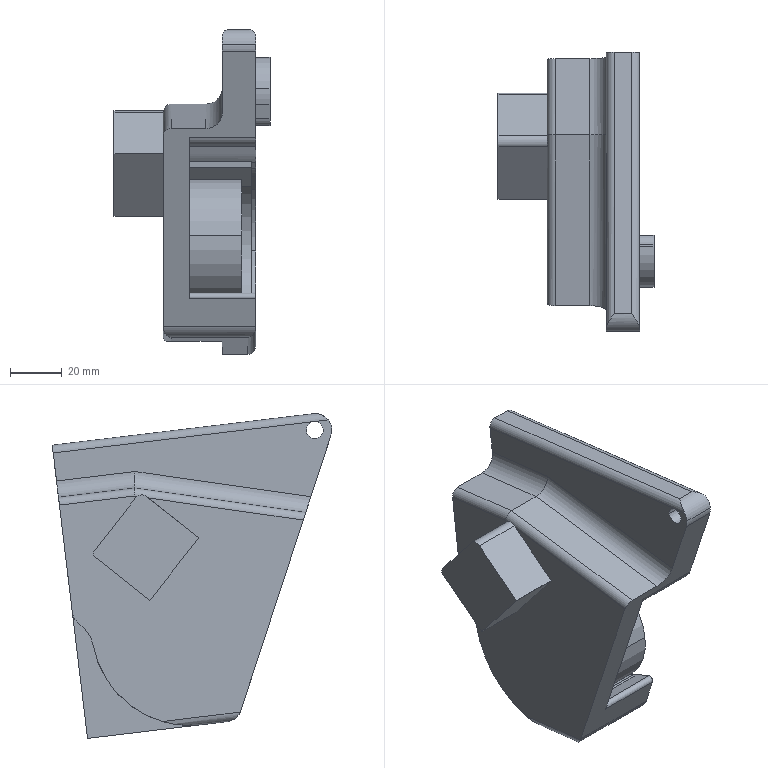Component | SolidWorks | DNR-71M20100BBEF2xx-A_500979-2 | 2 solids | 69 faces | volume 242640 mm3 | cylinder 36 | plane 33 | commonest cylinder face diameters 12.7 x6 6.081 x6 6.096 x3 49.337 x3 39.522 x2 52.121 x2 27.869 x2 6.528 x2